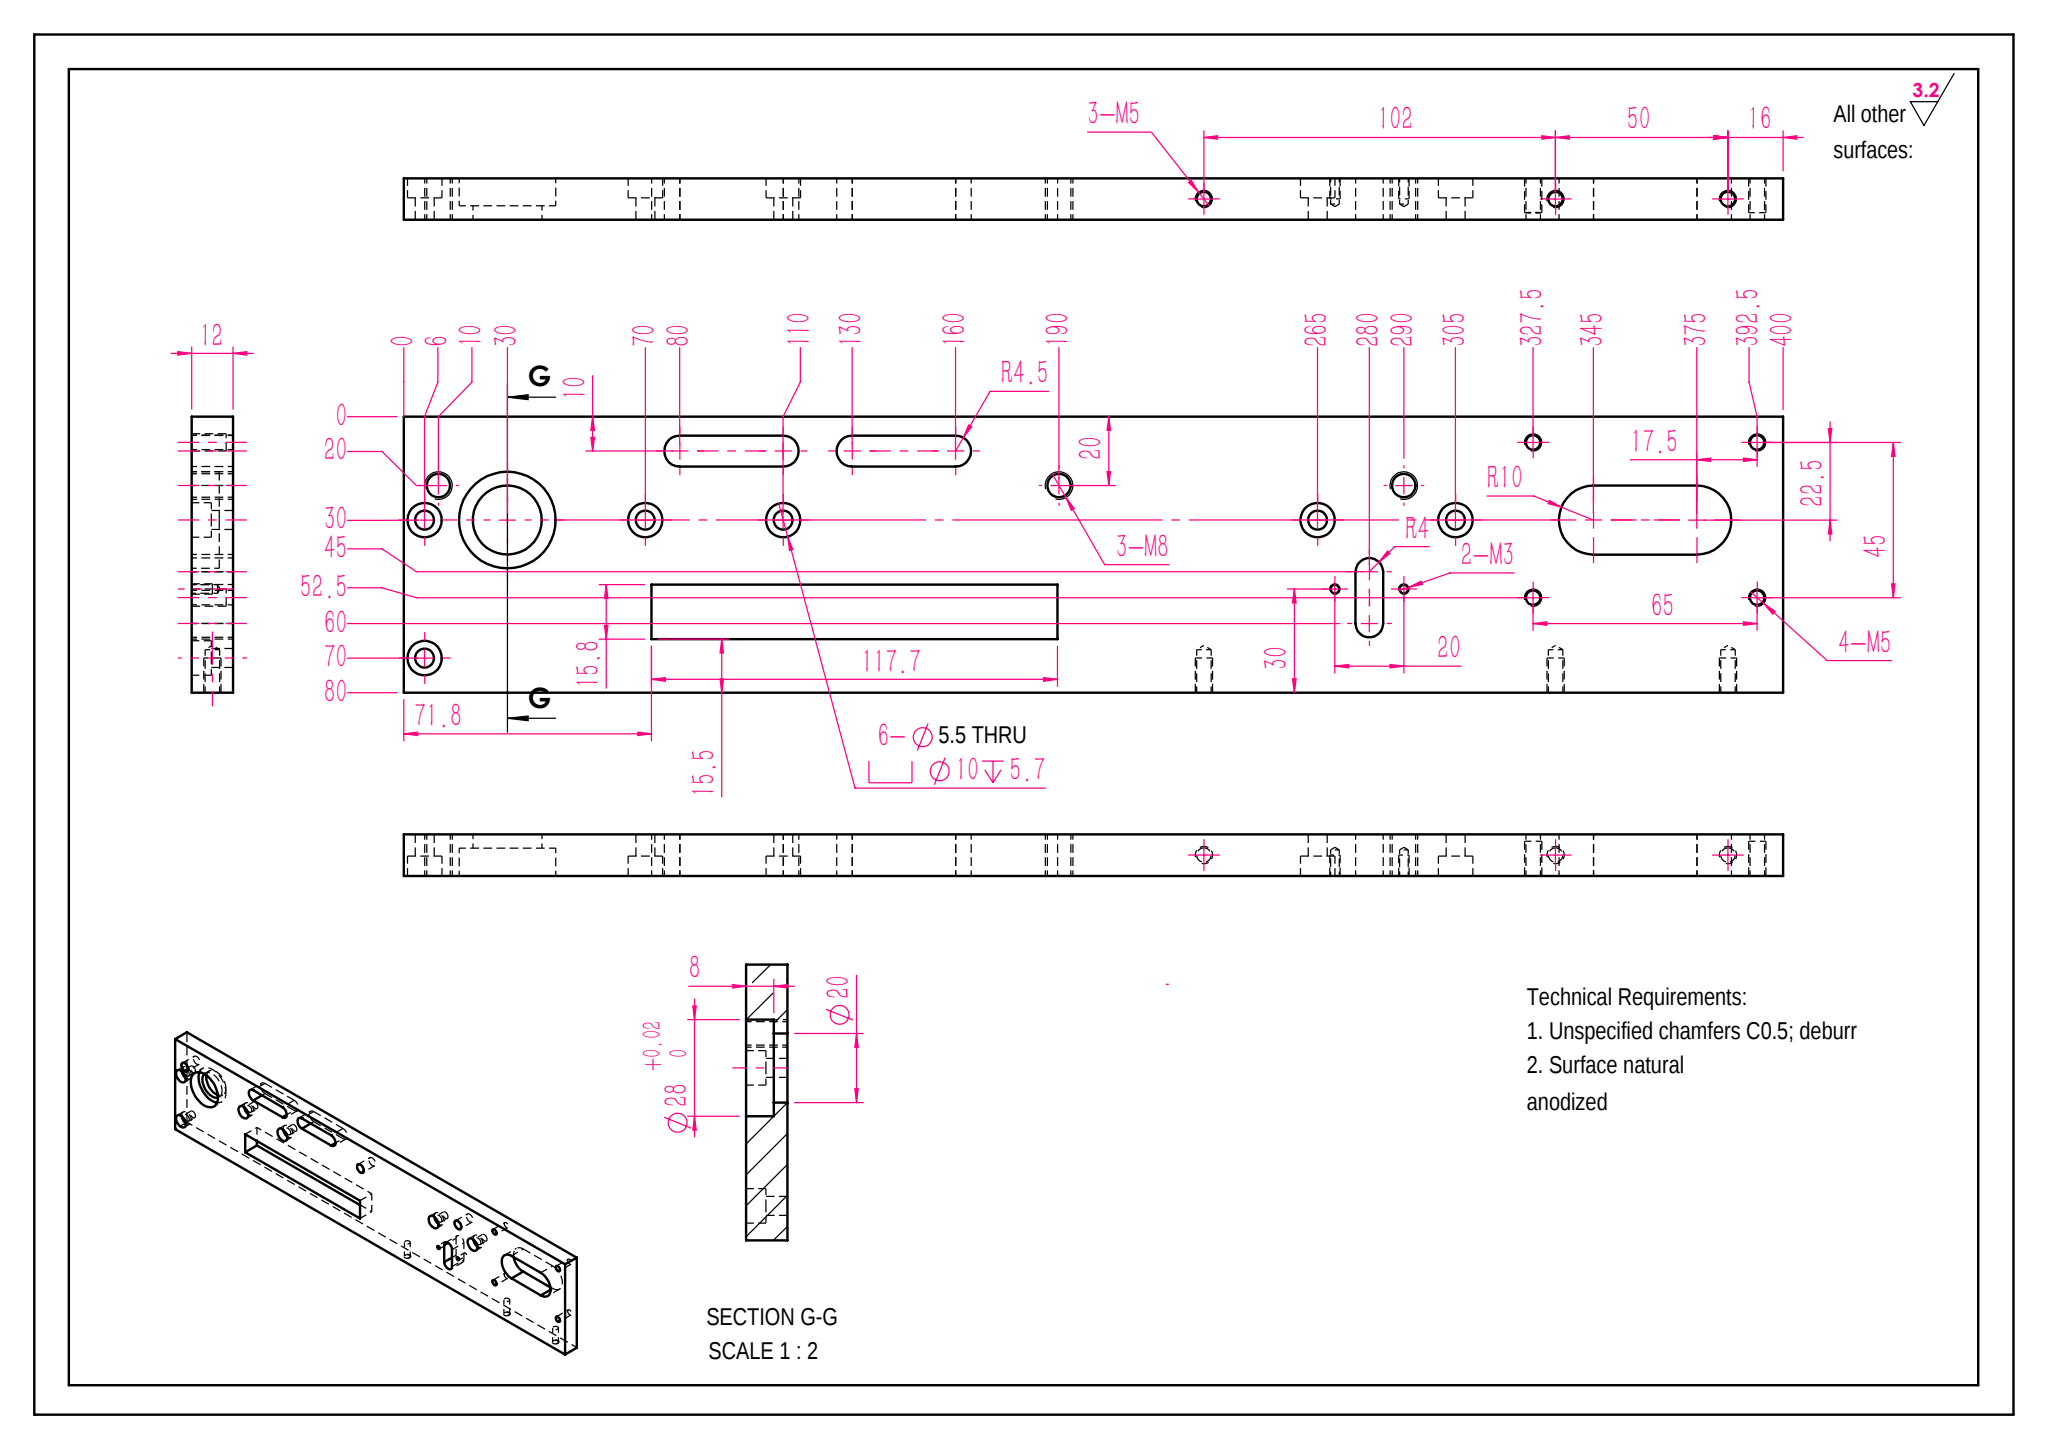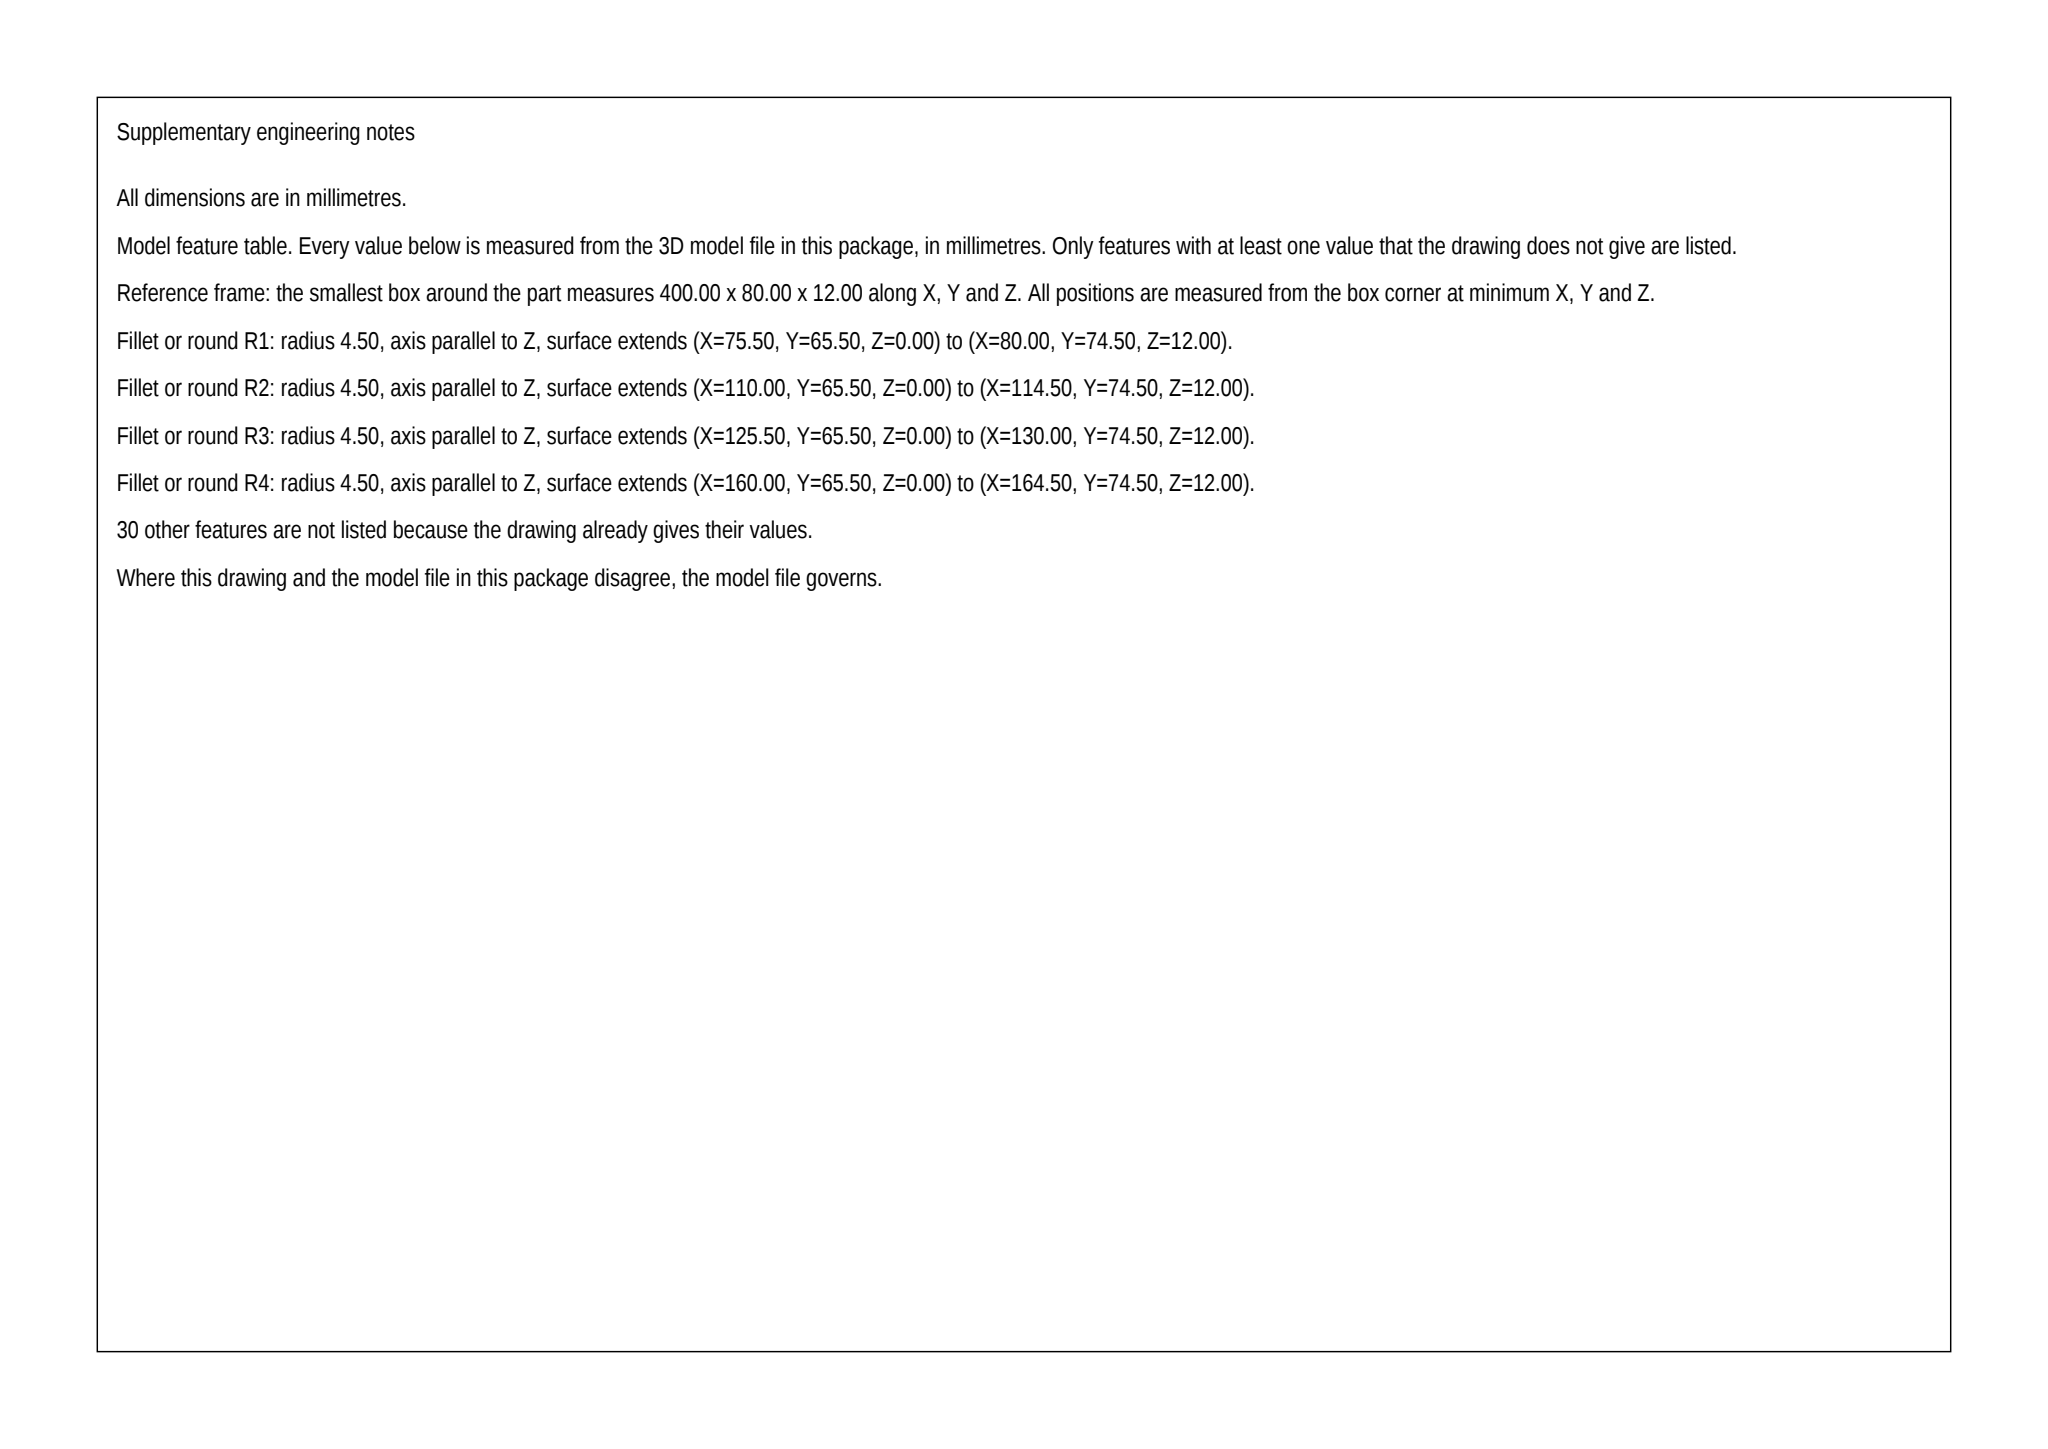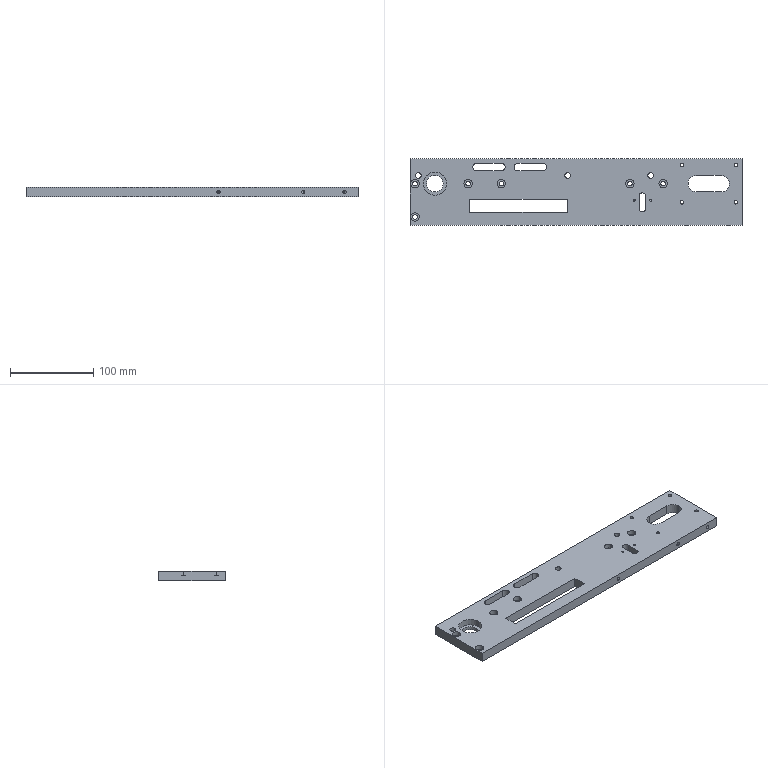Part | SolidWorks | mm | 1 solid | 98 faces | box 400 x 80 x 12 mm | volume 328272 mm3 | cylinder 63 | plane 25 | cone 10 | commonest cylinder face diameters 4.2 x14 10 x12 5.5 x12 9 x6 6.8 x6 20 x5 2.5 x4 28 x2
build123d program:
from build123d import *

# Parameters (mm, degrees)
SKETCH1_W                                            = 400
SKETCH1_H                                            = 80
BOSS_EXTRUDE1_DEPTH                                  = 12
SKETCH2_R                                            = 10
CUT_EXTRUDE1_DEPTH                                   = 205.313
SKETCH3_R                                            = 14
CUT_EXTRUDE2_DEPTH                                   = 8
M5_TAPPED_HOLE1_D                                    = 4.2
M5_TAPPED_HOLE1_DEPTH                                = 12.4
M5_TAPPED_HOLE1_TIP                                  = 1.262
HOLE_SIZE_ACCORDING_TO_HEXAGON_SOCKET_HE_D           = 5.5
HOLE_SIZE_ACCORDING_TO_HEXAGON_SOCKET_HE_CBORE_D     = 10
HOLE_SIZE_ACCORDING_TO_HEXAGON_SOCKET_HE_CBORE_DEPTH = 5.7
M8_TAPPED_HOLE1_D                                    = 6.8
M8_TAPPED_HOLE1_DEPTH                                = 19.75
M8_TAPPED_HOLE1_TIP                                  = 2.043
HOLE_SIZE_ACCORDING_TO_HEXAGON_SOCKE_2_D             = 5.5
HOLE_SIZE_ACCORDING_TO_HEXAGON_SOCKE_2_CBORE_D       = 10
HOLE_SIZE_ACCORDING_TO_HEXAGON_SOCKE_2_CBORE_DEPTH   = 5.7
CUT_EXTRUDE3_DEPTH                                   = 205.313
M3_TAPPED_HOLE1_D                                    = 2.5
M3_TAPPED_HOLE1_DEPTH                                = 7.5
M3_TAPPED_HOLE1_TIP                                  = 0.7511
CUT_EXTRUDE4_DEPTH                                   = 205.313
M5_TAPPED_HOLE2_D                                    = 4.2
M5_TAPPED_HOLE2_DEPTH                                = 12.4
M5_TAPPED_HOLE2_TIP                                  = 1.262
SKETCH20_W                                           = 117.742
SKETCH20_H                                           = 15.825
CUT_EXTRUDE5_DEPTH                                   = 71


with BuildPart() as part:
    # Sketch1 → Boss-Extrude1 (new body)
    with BuildSketch(Plane.XY):
        Rectangle(SKETCH1_W, SKETCH1_H)
    extrude(amount=BOSS_EXTRUDE1_DEPTH)

    # Sketch2 → Cut-Extrude1 (cut, through all)
    with BuildSketch(Plane.XY.offset(12)):
        with Locations((-170, 10)):
            Circle(SKETCH2_R)
        with BuildLine():
            Line((145, 20), (175, 20))
            ThreePointArc((175, 20), (185, 10), (175, 0))
            Line((175, 0), (145, 0))
            ThreePointArc((145, 0), (135, 10), (145, 20))
        make_face()
    extrude(amount=-CUT_EXTRUDE1_DEPTH, mode=Mode.SUBTRACT)

    # Sketch3 → Cut-Extrude2 (cut)
    with BuildSketch(Plane.XY.offset(12)):
        with Locations((-170, 10)):
            Circle(SKETCH3_R)
    extrude(amount=-CUT_EXTRUDE2_DEPTH, mode=Mode.SUBTRACT)

    # M5 Tapped Hole1
    with Locations(Plane.XY.offset(12)):
        with Locations((127.5, -12.5), (192.5, -12.5), (127.5, 32.5), (192.5, 32.5)):
            Hole(M5_TAPPED_HOLE1_D / 2, depth=M5_TAPPED_HOLE1_DEPTH)
            with Locations((0, 0, -(M5_TAPPED_HOLE1_DEPTH + M5_TAPPED_HOLE1_TIP / 2))):  # 118° drill point
                Cone(0, M5_TAPPED_HOLE1_D / 2, M5_TAPPED_HOLE1_TIP, mode=Mode.SUBTRACT)

    # Hole Size according to Hexagon Socket He (through all)
    with Locations(Plane.XY.offset(12)):
        with Locations((-130, 10), (-90, 10), (65, 10), (105, 10)):
            CounterBoreHole(HOLE_SIZE_ACCORDING_TO_HEXAGON_SOCKET_HE_D / 2, HOLE_SIZE_ACCORDING_TO_HEXAGON_SOCKET_HE_CBORE_D / 2, HOLE_SIZE_ACCORDING_TO_HEXAGON_SOCKET_HE_CBORE_DEPTH)

    # M8 Tapped Hole1
    with Locations(Plane.XY.offset(12)):
        with Locations((90, 20), (-10, 20), (-190, 20)):
            Hole(M8_TAPPED_HOLE1_D / 2, depth=M8_TAPPED_HOLE1_DEPTH)
            with Locations((0, 0, -(M8_TAPPED_HOLE1_DEPTH + M8_TAPPED_HOLE1_TIP / 2))):  # 118° drill point
                Cone(0, M8_TAPPED_HOLE1_D / 2, M8_TAPPED_HOLE1_TIP, mode=Mode.SUBTRACT)

    # Hole Size according to Hexagon Socke 2 (through all)
    with Locations(Plane.XY.offset(12)):
        with Locations((-194, -30), (-194, 10)):
            CounterBoreHole(HOLE_SIZE_ACCORDING_TO_HEXAGON_SOCKE_2_D / 2, HOLE_SIZE_ACCORDING_TO_HEXAGON_SOCKE_2_CBORE_D / 2, HOLE_SIZE_ACCORDING_TO_HEXAGON_SOCKE_2_CBORE_DEPTH)

    # Sketch14 → Cut-Extrude3 (cut, through all)
    with BuildSketch(Plane.XY.offset(12)):
        with BuildLine():
            Line((84, -5), (84, -20))
            ThreePointArc((84, -20), (80, -24), (76, -20))
            Line((76, -20), (76, -5))
            ThreePointArc((76, -5), (80, -1), (84, -5))
        make_face()
    extrude(amount=-CUT_EXTRUDE3_DEPTH, mode=Mode.SUBTRACT)

    # M3 Tapped Hole1
    with Locations(Plane.XY.offset(12)):
        with Locations((90, -10), (70, -10)):
            Hole(M3_TAPPED_HOLE1_D / 2, depth=M3_TAPPED_HOLE1_DEPTH)
            with Locations((0, 0, -(M3_TAPPED_HOLE1_DEPTH + M3_TAPPED_HOLE1_TIP / 2))):  # 118° drill point
                Cone(0, M3_TAPPED_HOLE1_D / 2, M3_TAPPED_HOLE1_TIP, mode=Mode.SUBTRACT)

    # Sketch17 → Cut-Extrude4 (cut, through all)
    with BuildSketch(Plane(origin=(0, 0, 0), x_dir=(-1, 0, 0), z_dir=(0, 0, -1))):
        with BuildLine():
            Line((40, 34.5), (70, 34.5))
            ThreePointArc((70, 34.5), (74.5, 30), (70, 25.5))
            Line((70, 25.5), (40, 25.5))
            ThreePointArc((40, 25.5), (35.5, 30), (40, 34.5))
        make_face()
        with BuildLine():
            Line((90, 34.5), (120, 34.5))
            ThreePointArc((120, 34.5), (124.5, 30), (120, 25.5))
            Line((120, 25.5), (90, 25.5))
            ThreePointArc((90, 25.5), (85.5, 30), (90, 34.5))
        make_face()
    extrude(amount=-CUT_EXTRUDE4_DEPTH, mode=Mode.SUBTRACT)

    # M5 Tapped Hole2
    with Locations(Plane(origin=(0, -40, 0), x_dir=(-1, 0, 0), z_dir=(0, -1, 0))):
        with Locations((-32, -6), (-184, -6), (-134, -6)):
            Hole(M5_TAPPED_HOLE2_D / 2, depth=M5_TAPPED_HOLE2_DEPTH)
            with Locations((0, 0, -(M5_TAPPED_HOLE2_DEPTH + M5_TAPPED_HOLE2_TIP / 2))):  # 118° drill point
                Cone(0, M5_TAPPED_HOLE2_D / 2, M5_TAPPED_HOLE2_TIP, mode=Mode.SUBTRACT)

    # Sketch20 → Cut-Extrude5 (cut)
    with BuildSketch(Plane.XY.offset(12)):
        with Locations((-69.316, -16.617)):
            Rectangle(SKETCH20_W, SKETCH20_H)
    extrude(amount=-CUT_EXTRUDE5_DEPTH, mode=Mode.SUBTRACT)


solid = part.part